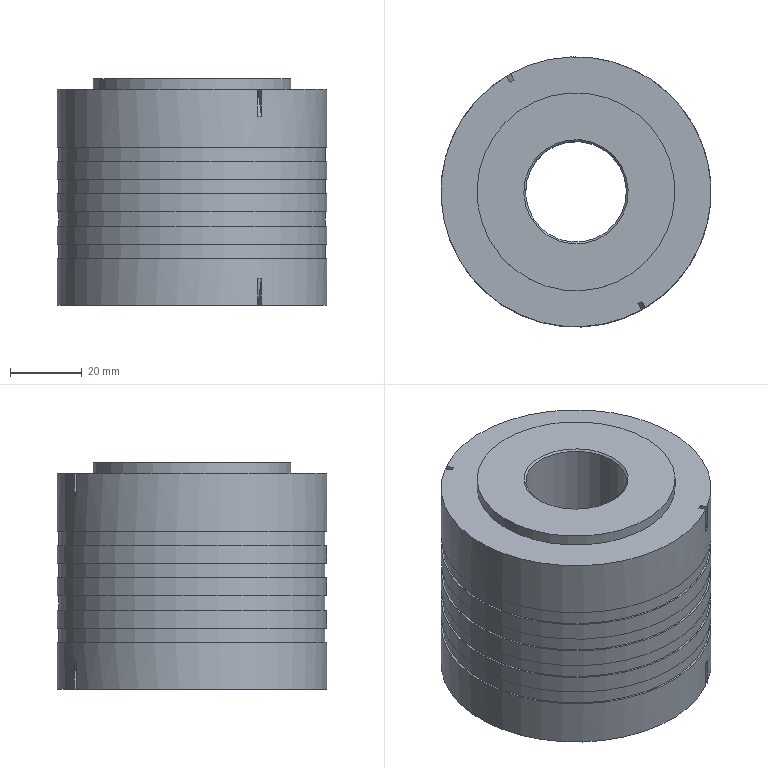Component | NX | PISTON | 1 solid | 38 faces | volume 197780 mm3 | plane 20 | cylinder 12 | cone 6 | commonest cylinder face diameters 75 x5 74 x4 55 x1 50 x1 28 x1